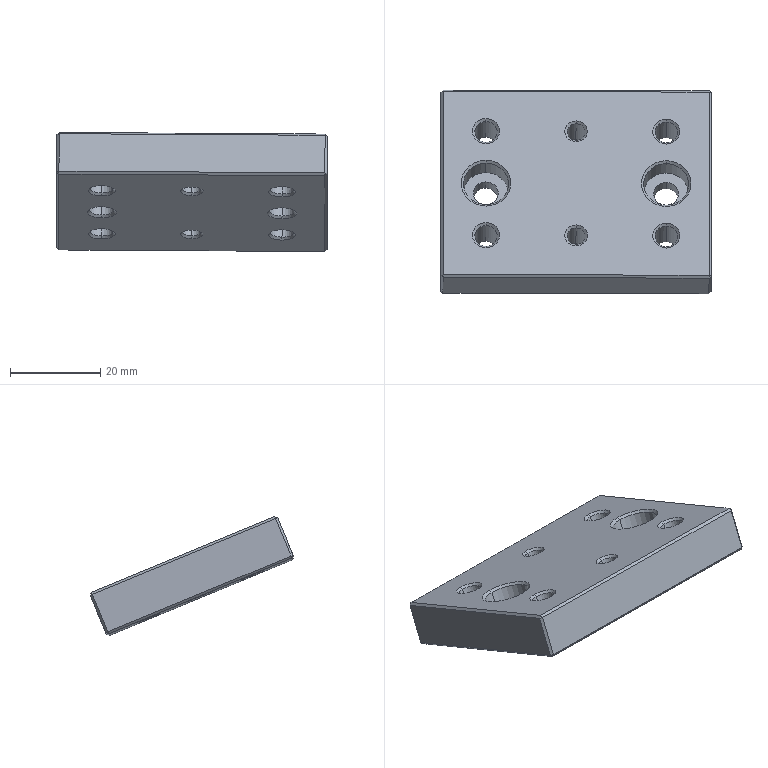Component | SolidWorks | 11-1 | 1 solid | 80 faces | box 60.06 x 45.16 x 26.42 mm | volume 24749 mm3 | cone 32 | plane 28 | cylinder 20 | commonest cylinder face diameters 5 x8 4 x4 10 x4 5.5 x4
build123d program:
from build123d import *

# Parameters (mm, degrees)
SKETCH1_W                                       = 45
SKETCH1_H                                       = 60
BOSS_EXTRUDE1_DEPTH                             = 10
M6_TAPPED_HOLE1_D                               = 5
M6_TAPPED_HOLE1_DEPTH                           = 15
M6_TAPPED_HOLE1_TIP                             = 1.502
M5_HEX_SOCKET_HEAD_CAP_SCREW_CBORE1_D           = 5.5
M5_HEX_SOCKET_HEAD_CAP_SCREW_CBORE1_CBORE_D     = 10
M5_HEX_SOCKET_HEAD_CAP_SCREW_CBORE1_CBORE_DEPTH = 5.9
SIZE_MM_DOWEL_PIN_HOLE2_D                       = 4
SIZE_MM_DOWEL_PIN_HOLE2_DEPTH                   = 10
SIZE_MM_DOWEL_PIN_HOLE2_TIP                     = 1.202
CHAMFER1_SIZE                                   = 0.5


with BuildPart() as part:
    # Sketch1 → Boss-Extrude1 (new body)
    with BuildSketch(Plane.XY):
        Rectangle(SKETCH1_W, SKETCH1_H)
    extrude(amount=BOSS_EXTRUDE1_DEPTH)

    # M6 Tapped Hole1
    with Locations(Plane.XY.offset(10)):
        with Locations((12.5, -20), (-12.5, 20), (-12.5, -20), (12.5, 20)):
            Hole(M6_TAPPED_HOLE1_D / 2, depth=M6_TAPPED_HOLE1_DEPTH)
            with Locations((0, 0, -(M6_TAPPED_HOLE1_DEPTH + M6_TAPPED_HOLE1_TIP / 2))):  # 118° drill point
                Cone(0, M6_TAPPED_HOLE1_D / 2, M6_TAPPED_HOLE1_TIP, mode=Mode.SUBTRACT)

    # M5 Hex Socket Head Cap Screw CBORE1 (through all)
    with Locations(Plane.XY.offset(10)):
        with Locations((0, 20), (0, -20)):
            CounterBoreHole(M5_HEX_SOCKET_HEAD_CAP_SCREW_CBORE1_D / 2, M5_HEX_SOCKET_HEAD_CAP_SCREW_CBORE1_CBORE_D / 2, M5_HEX_SOCKET_HEAD_CAP_SCREW_CBORE1_CBORE_DEPTH)

    # Size mm Dowel Pin Hole2
    with Locations(Plane.XY.offset(10)):
        with Locations((-12.5, 0), (12.5, 0)):
            Hole(SIZE_MM_DOWEL_PIN_HOLE2_D / 2, depth=SIZE_MM_DOWEL_PIN_HOLE2_DEPTH)
            with Locations((0, 0, -(SIZE_MM_DOWEL_PIN_HOLE2_DEPTH + SIZE_MM_DOWEL_PIN_HOLE2_TIP / 2))):  # 118° drill point
                Cone(0, SIZE_MM_DOWEL_PIN_HOLE2_D / 2, SIZE_MM_DOWEL_PIN_HOLE2_TIP, mode=Mode.SUBTRACT)

    # Chamfer1
    chamfer1_edges = [part.edges().sort_by_distance(p)[0] for p in [
        (-22.5, 0, 10),
        (0, -30, 10),
        (15, 20, 0),
        (15, 20, 10),
        (-10, -20, 0),
        (-10, -20, 10),
        (-10, 20, 0),
        (-10, 20, 10),
        (15, -20, 0),
        (15, -20, 10),
        (22.5, 0, 10),
        (-5, -20, 10),
        (2.75, -20, 0),
        (0, -30, 0),
        (-5, 20, 10),
        (2.75, 20, 0),
        (-22.5, 0, 0),
        (0, 30, 0),
        (14.5, 0, 10),
        (14.5, 0, 0),
        (22.5, 0, 0),
        (-10.5, 0, 10),
        (-10.5, 0, 0),
        (0, 30, 10),
        (22.5, -30, 5),
        (-22.5, -30, 5),
        (-22.5, 30, 5),
        (22.5, 30, 5),
    ]]
    chamfer(chamfer1_edges, length=CHAMFER1_SIZE)


solid = part.part

# Placed as in the assembly
solid = solid.moved(Location((104.012, -68.459, 468.513), (-22.484, 0.3658, -89.992)))